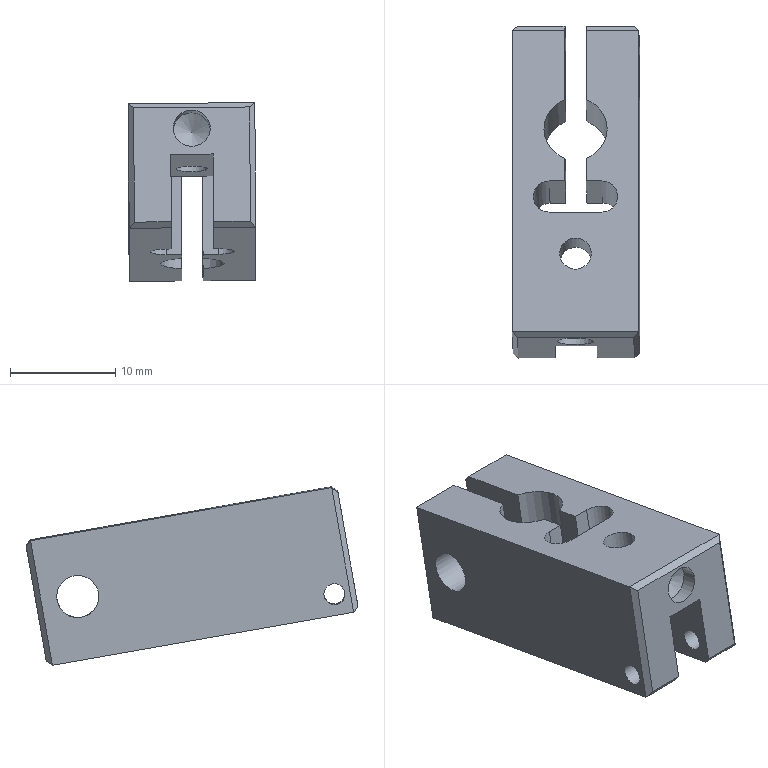Component | NX | INDICATOR_CLAMP_BLOCK | 1 solid | 41 faces | volume 2939 mm3 | plane 29 | cylinder 10 | cone 2 | commonest cylinder face diameters 3 x3 6 x2 2 x2 3.5 x1 4.2 x1 4 x1